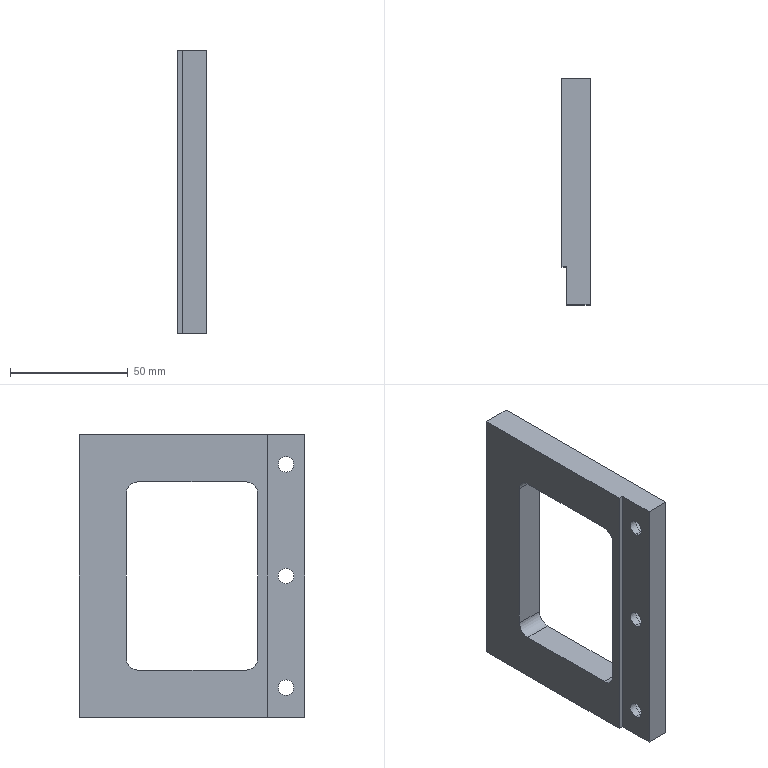Component | SolidWorks | F01AE00111-A2015-1 | 1 solid | 43 faces | box 12 x 96 x 120 mm | volume 77717 mm3 | cylinder 22 | plane 15 | cone 6 | commonest cylinder face diameters 5 x6 11 x6 6.6 x6 10 x4
build123d program:
from build123d import *

# Parameters (mm, degrees)
SKETCH1_W                                            = 120
SKETCH1_H                                            = 96
BOSS_EXTRUDE1_DEPTH                                  = 12
SKETCH2_W                                            = 80
SKETCH2_H                                            = 56
CUT_EXTRUDE1_DEPTH                                   = 78.769
FILLET1_R                                            = 5
SKETCH3_W                                            = 120
SKETCH3_H                                            = 16
CUT_EXTRUDE2_DEPTH                                   = 2
HOLE_SIZE_ACCORDING_TO_THE_TYPE_1_OF_HEX_D           = 6.6
HOLE_SIZE_ACCORDING_TO_THE_TYPE_1_OF_HEX_CBORE_D     = 11
HOLE_SIZE_ACCORDING_TO_THE_TYPE_1_OF_HEX_CBORE_DEPTH = 6.8
M6_TAPPED_HOLE1_D                                    = 5
M6_TAPPED_HOLE1_DEPTH                                = 15
M6_TAPPED_HOLE1_TIP                                  = 1.502


with BuildPart() as part:
    # Sketch1 → Boss-Extrude1 (new body)
    with BuildSketch(Plane.XY):
        Rectangle(SKETCH1_W, SKETCH1_H)
    extrude(amount=BOSS_EXTRUDE1_DEPTH)

    # Sketch2 → Cut-Extrude1 (cut, through all)
    with BuildSketch(Plane.XY.offset(12)):
        Rectangle(SKETCH2_W, SKETCH2_H)
    extrude(amount=-CUT_EXTRUDE1_DEPTH, mode=Mode.SUBTRACT)

    # Fillet1
    fillet1_edges = [part.edges().sort_by_distance(p)[0] for p in [
        (40, 28, 6),
        (40, -28, 6),
        (-40, -28, 6),
        (-40, 28, 6),
    ]]
    fillet(fillet1_edges, radius=FILLET1_R)

    # Sketch3 → Cut-Extrude2 (cut)
    with BuildSketch(Plane.XY.offset(12)):
        with Locations((0, -40)):
            Rectangle(SKETCH3_W, SKETCH3_H)
    extrude(amount=-CUT_EXTRUDE2_DEPTH, mode=Mode.SUBTRACT)

    # Hole size according to the type 1 of hex (through all)
    with Locations(Plane(origin=(0, 0, 0), x_dir=(-1, 0, 0), z_dir=(0, 0, -1))):
        with Locations((-47.5, -40), (0, -40), (47.5, -40)):
            CounterBoreHole(HOLE_SIZE_ACCORDING_TO_THE_TYPE_1_OF_HEX_D / 2, HOLE_SIZE_ACCORDING_TO_THE_TYPE_1_OF_HEX_CBORE_D / 2, HOLE_SIZE_ACCORDING_TO_THE_TYPE_1_OF_HEX_CBORE_DEPTH)

    # M6 Tapped Hole1
    with Locations(Plane(origin=(0, 48, 0), x_dir=(1, 0, 0), z_dir=(0, 1, 0))):
        with Locations((-47.5, -6), (0, -6), (47.5, -6)):
            Hole(M6_TAPPED_HOLE1_D / 2, depth=M6_TAPPED_HOLE1_DEPTH)
            with Locations((0, 0, -(M6_TAPPED_HOLE1_DEPTH + M6_TAPPED_HOLE1_TIP / 2))):  # 118° drill point
                Cone(0, M6_TAPPED_HOLE1_D / 2, M6_TAPPED_HOLE1_TIP, mode=Mode.SUBTRACT)


solid = part.part

# Placed as in the assembly
solid = solid.moved(Location((-34.352, 44.548, -252.975), (0, -90, 0)))